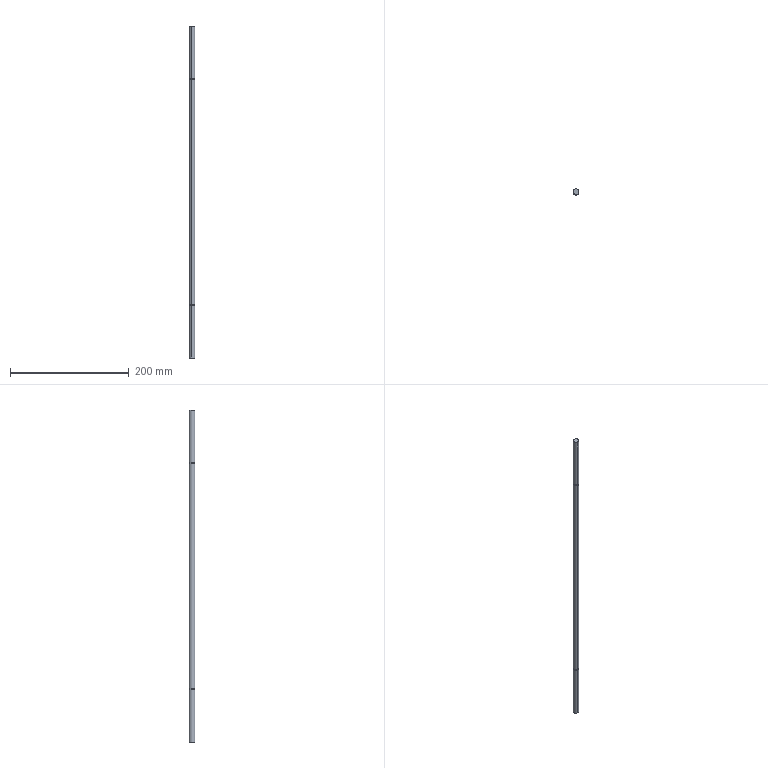Component | SolidWorks | FilmGuideRodAxis-1 | 1 solid | 16 faces | box 10 x 10 x 559 mm | volume 43894 mm3 | cylinder 10 | plane 6 | commonest cylinder face diameters 10 x6 9.7 x4
build123d program:
from build123d import *


with BuildPart() as part:
    # Sketch1 → Revolve1 (revolve)
    with BuildSketch(Plane(origin=(0, 0, 0), x_dir=(-1, 0, 0), z_dir=(0, 0, -1)), mode=Mode.PRIVATE) as revolve1_sk:
        Polygon((-279.5, 5), (-279.5, 0), (279.5, 0), (279.5, 5), (191.1, 5), (191.1, 4.85), (190, 4.85), (190, 5), (-190, 5), (-190, 4.85), (-191.1, 4.85), (-191.1, 5), align=None)
    revolve(revolve1_sk.sketch.rotate(Axis((279.5, 0, 0), (-1, 0, 0)), 270), axis=Axis((279.5, 0, 0), (-1, 0, 0)))


solid = part.part

# Placed as in the assembly
solid = solid.moved(Location((376.258, 489.105, 0), (0, 90, 0)))
STEP:
#1=CARTESIAN_POINT('',(14.853,19.443,7.524));
#2=VERTEX_POINT('',#1);
#3=CARTESIAN_POINT('',(14.773,19.069,7.524));
#4=VERTEX_POINT('',#3);
#5=CARTESIAN_POINT('',(14.813,19.256,7.524));
#6=DIRECTION('',(0.,-0.,-1.));
#7=DIRECTION('',(0.2099,0.9777,0.));
#8=AXIS2_PLACEMENT_3D('',#5,#6,#7);
#9=CIRCLE('',#8,0.1909);
#10=EDGE_CURVE('',#2,#4,#9,.T.);
#11=ORIENTED_EDGE('',*,*,#10,.T.);
#12=CARTESIAN_POINT('',(14.773,19.069,7.48));
#13=VERTEX_POINT('',#12);
#14=CARTESIAN_POINT('',(14.773,19.069,11.004));
#15=DIRECTION('',(0.,-0.,-1.));
#16=VECTOR('',#15,39.37);
#17=LINE('',#14,#16);
#18=EDGE_CURVE('',#4,#13,#17,.T.);
#19=ORIENTED_EDGE('',*,*,#18,.T.);
#20=CARTESIAN_POINT('',(14.853,19.443,7.48));
#21=VERTEX_POINT('',#20);
#22=CARTESIAN_POINT('',(14.813,19.256,7.48));
#23=DIRECTION('',(0.,-0.,-1.));
#24=DIRECTION('',(0.2099,0.9777,0.));
#25=AXIS2_PLACEMENT_3D('',#22,#23,#24);
#26=CIRCLE('',#25,0.1909);
#27=EDGE_CURVE('',#21,#13,#26,.T.);
#28=ORIENTED_EDGE('',*,*,#27,.F.);
#29=CARTESIAN_POINT('',(14.853,19.443,11.004));
#30=DIRECTION('',(0.,-0.,-1.));
#31=VECTOR('',#30,39.37);
#32=LINE('',#29,#31);
#33=EDGE_CURVE('',#2,#21,#32,.T.);
#34=ORIENTED_EDGE('',*,*,#33,.F.);
#35=EDGE_LOOP('',(#11,#19,#28,#34));
#36=FACE_OUTER_BOUND('',#35,.T.);
#37=CARTESIAN_POINT('',(14.813,19.256,11.004));
#38=DIRECTION('',(0.,-0.,-1.));
#39=DIRECTION('',(0.2099,0.9777,0.));
#40=AXIS2_PLACEMENT_3D('',#37,#38,#39);
#41=CYLINDRICAL_SURFACE('',#40,0.1909);
#42=ADVANCED_FACE('',(#36),#41,.T.);
#43=CARTESIAN_POINT('',(14.855,19.449,7.48));
#44=VERTEX_POINT('',#43);
#45=CARTESIAN_POINT('',(14.772,19.064,7.48));
#46=VERTEX_POINT('',#45);
#47=CARTESIAN_POINT('',(14.813,19.256,7.48));
#48=DIRECTION('',(0.,-0.,-1.));
#49=DIRECTION('',(0.2099,0.9777,0.));
#50=AXIS2_PLACEMENT_3D('',#47,#48,#49);
#51=CIRCLE('',#50,0.1969);
#52=EDGE_CURVE('',#44,#46,#51,.T.);
#53=ORIENTED_EDGE('',*,*,#52,.T.);
#54=CARTESIAN_POINT('',(14.772,19.064,-7.48));
#55=VERTEX_POINT('',#54);
#56=CARTESIAN_POINT('',(14.772,19.064,11.004));
#57=DIRECTION('',(0.,-0.,-1.));
#58=VECTOR('',#57,39.37);
#59=LINE('',#56,#58);
#60=EDGE_CURVE('',#46,#55,#59,.T.);
#61=ORIENTED_EDGE('',*,*,#60,.T.);
#62=CARTESIAN_POINT('',(14.855,19.449,-7.48));
#63=VERTEX_POINT('',#62);
#64=CARTESIAN_POINT('',(14.813,19.256,-7.48));
#65=DIRECTION('',(0.,-0.,-1.));
#66=DIRECTION('',(0.2099,0.9777,0.));
#67=AXIS2_PLACEMENT_3D('',#64,#65,#66);
#68=CIRCLE('',#67,0.1969);
#69=EDGE_CURVE('',#63,#55,#68,.T.);
#70=ORIENTED_EDGE('',*,*,#69,.F.);
#71=CARTESIAN_POINT('',(14.855,19.449,11.004));
#72=DIRECTION('',(0.,-0.,-1.));
#73=VECTOR('',#72,39.37);
#74=LINE('',#71,#73);
#75=EDGE_CURVE('',#44,#63,#74,.T.);
#76=ORIENTED_EDGE('',*,*,#75,.F.);
#77=EDGE_LOOP('',(#53,#61,#70,#76));
#78=FACE_OUTER_BOUND('',#77,.T.);
#79=CARTESIAN_POINT('',(14.813,19.256,11.004));
#80=DIRECTION('',(0.,-0.,-1.));
#81=DIRECTION('',(0.2099,0.9777,0.));
#82=AXIS2_PLACEMENT_3D('',#79,#80,#81);
#83=CYLINDRICAL_SURFACE('',#82,0.1969);
#84=ADVANCED_FACE('',(#78),#83,.T.);
#85=CARTESIAN_POINT('',(14.853,19.443,-7.48));
#86=VERTEX_POINT('',#85);
#87=CARTESIAN_POINT('',(14.773,19.069,-7.48));
#88=VERTEX_POINT('',#87);
#89=CARTESIAN_POINT('',(14.813,19.256,-7.48));
#90=DIRECTION('',(0.,-0.,-1.));
#91=DIRECTION('',(0.2099,0.9777,0.));
#92=AXIS2_PLACEMENT_3D('',#89,#90,#91);
#93=CIRCLE('',#92,0.1909);
#94=EDGE_CURVE('',#86,#88,#93,.T.);
#95=ORIENTED_EDGE('',*,*,#94,.T.);
#96=CARTESIAN_POINT('',(14.773,19.069,-7.524));
#97=VERTEX_POINT('',#96);
#98=CARTESIAN_POINT('',(14.773,19.069,11.004));
#99=DIRECTION('',(0.,-0.,-1.));
#100=VECTOR('',#99,39.37);
#101=LINE('',#98,#100);
#102=EDGE_CURVE('',#88,#97,#101,.T.);
#103=ORIENTED_EDGE('',*,*,#102,.T.);
#104=CARTESIAN_POINT('',(14.853,19.443,-7.524));
#105=VERTEX_POINT('',#104);
#106=CARTESIAN_POINT('',(14.813,19.256,-7.524));
#107=DIRECTION('',(0.,-0.,-1.));
#108=DIRECTION('',(0.2099,0.9777,0.));
#109=AXIS2_PLACEMENT_3D('',#106,#107,#108);
#110=CIRCLE('',#109,0.1909);
#111=EDGE_CURVE('',#105,#97,#110,.T.);
#112=ORIENTED_EDGE('',*,*,#111,.F.);
#113=CARTESIAN_POINT('',(14.853,19.443,11.004));
#114=DIRECTION('',(0.,-0.,-1.));
#115=VECTOR('',#114,39.37);
#116=LINE('',#113,#115);
#117=EDGE_CURVE('',#86,#105,#116,.T.);
#118=ORIENTED_EDGE('',*,*,#117,.F.);
#119=EDGE_LOOP('',(#95,#103,#112,#118));
#120=FACE_OUTER_BOUND('',#119,.T.);
#121=CARTESIAN_POINT('',(14.813,19.256,11.004));
#122=DIRECTION('',(0.,-0.,-1.));
#123=DIRECTION('',(0.2099,0.9777,0.));
#124=AXIS2_PLACEMENT_3D('',#121,#122,#123);
#125=CYLINDRICAL_SURFACE('',#124,0.1909);
#126=ADVANCED_FACE('',(#120),#125,.T.);
#127=CARTESIAN_POINT('',(14.855,19.449,-7.524));
#128=VERTEX_POINT('',#127);
#129=CARTESIAN_POINT('',(14.772,19.064,-7.524));
#130=VERTEX_POINT('',#129);
#131=CARTESIAN_POINT('',(14.813,19.256,-7.524));
#132=DIRECTION('',(0.,-0.,-1.));
#133=DIRECTION('',(0.2099,0.9777,0.));
#134=AXIS2_PLACEMENT_3D('',#131,#132,#133);
#135=CIRCLE('',#134,0.1969);
#136=EDGE_CURVE('',#128,#130,#135,.T.);
#137=ORIENTED_EDGE('',*,*,#136,.T.);
#138=CARTESIAN_POINT('',(14.772,19.064,-11.004));
#139=VERTEX_POINT('',#138);
#140=CARTESIAN_POINT('',(14.772,19.064,11.004));
#141=DIRECTION('',(0.,-0.,-1.));
#142=VECTOR('',#141,39.37);
#143=LINE('',#140,#142);
#144=EDGE_CURVE('',#130,#139,#143,.T.);
#145=ORIENTED_EDGE('',*,*,#144,.T.);
#146=CARTESIAN_POINT('',(14.855,19.449,-11.004));
#147=VERTEX_POINT('',#146);
#148=CARTESIAN_POINT('',(14.813,19.256,-11.004));
#149=DIRECTION('',(0.,-0.,-1.));
#150=DIRECTION('',(0.2099,0.9777,0.));
#151=AXIS2_PLACEMENT_3D('',#148,#149,#150);
#152=CIRCLE('',#151,0.1969);
#153=EDGE_CURVE('',#147,#139,#152,.T.);
#154=ORIENTED_EDGE('',*,*,#153,.F.);
#155=CARTESIAN_POINT('',(14.855,19.449,11.004));
#156=DIRECTION('',(0.,-0.,-1.));
#157=VECTOR('',#156,39.37);
#158=LINE('',#155,#157);
#159=EDGE_CURVE('',#128,#147,#158,.T.);
#160=ORIENTED_EDGE('',*,*,#159,.F.);
#161=EDGE_LOOP('',(#137,#145,#154,#160));
#162=FACE_OUTER_BOUND('',#161,.T.);
#163=CARTESIAN_POINT('',(14.813,19.256,11.004));
#164=DIRECTION('',(0.,-0.,-1.));
#165=DIRECTION('',(0.2099,0.9777,0.));
#166=AXIS2_PLACEMENT_3D('',#163,#164,#165);
#167=CYLINDRICAL_SURFACE('',#166,0.1969);
#168=ADVANCED_FACE('',(#162),#167,.T.);
#169=CARTESIAN_POINT('',(14.855,19.449,11.004));
#170=VERTEX_POINT('',#169);
#171=CARTESIAN_POINT('',(14.772,19.064,11.004));
#172=VERTEX_POINT('',#171);
#173=CARTESIAN_POINT('',(14.813,19.256,11.004));
#174=DIRECTION('',(0.,-0.,-1.));
#175=DIRECTION('',(0.2099,0.9777,0.));
#176=AXIS2_PLACEMENT_3D('',#173,#174,#175);
#177=CIRCLE('',#176,0.1969);
#178=EDGE_CURVE('',#170,#172,#177,.T.);
#179=ORIENTED_EDGE('',*,*,#178,.T.);
#180=CARTESIAN_POINT('',(14.772,19.064,7.524));
#181=VERTEX_POINT('',#180);
#182=CARTESIAN_POINT('',(14.772,19.064,11.004));
#183=DIRECTION('',(0.,-0.,-1.));
#184=VECTOR('',#183,39.37);
#185=LINE('',#182,#184);
#186=EDGE_CURVE('',#172,#181,#185,.T.);
#187=ORIENTED_EDGE('',*,*,#186,.T.);
#188=CARTESIAN_POINT('',(14.855,19.449,7.524));
#189=VERTEX_POINT('',#188);
#190=CARTESIAN_POINT('',(14.813,19.256,7.524));
#191=DIRECTION('',(0.,-0.,-1.));
#192=DIRECTION('',(0.2099,0.9777,0.));
#193=AXIS2_PLACEMENT_3D('',#190,#191,#192);
#194=CIRCLE('',#193,0.1969);
#195=EDGE_CURVE('',#189,#181,#194,.T.);
#196=ORIENTED_EDGE('',*,*,#195,.F.);
#197=CARTESIAN_POINT('',(14.855,19.449,11.004));
#198=DIRECTION('',(0.,-0.,-1.));
#199=VECTOR('',#198,39.37);
#200=LINE('',#197,#199);
#201=EDGE_CURVE('',#170,#189,#200,.T.);
#202=ORIENTED_EDGE('',*,*,#201,.F.);
#203=EDGE_LOOP('',(#179,#187,#196,#202));
#204=FACE_OUTER_BOUND('',#203,.T.);
#205=CARTESIAN_POINT('',(14.813,19.256,11.004));
#206=DIRECTION('',(0.,-0.,-1.));
#207=DIRECTION('',(0.2099,0.9777,0.));
#208=AXIS2_PLACEMENT_3D('',#205,#206,#207);
#209=CYLINDRICAL_SURFACE('',#208,0.1969);
#210=ADVANCED_FACE('',(#204),#209,.T.);
#211=ORIENTED_EDGE('',*,*,#186,.F.);
#212=CARTESIAN_POINT('',(14.813,19.256,11.004));
#213=DIRECTION('',(0.,-0.,-1.));
#214=DIRECTION('',(0.2099,0.9777,0.));
#215=AXIS2_PLACEMENT_3D('',#212,#213,#214);
#216=CIRCLE('',#215,0.1969);
#217=EDGE_CURVE('',#172,#170,#216,.T.);
#218=ORIENTED_EDGE('',*,*,#217,.T.);
#219=ORIENTED_EDGE('',*,*,#201,.T.);
#220=CARTESIAN_POINT('',(14.813,19.256,7.524));
#221=DIRECTION('',(0.,-0.,-1.));
#222=DIRECTION('',(0.2099,0.9777,0.));
#223=AXIS2_PLACEMENT_3D('',#220,#221,#222);
#224=CIRCLE('',#223,0.1969);
#225=EDGE_CURVE('',#181,#189,#224,.T.);
#226=ORIENTED_EDGE('',*,*,#225,.F.);
#227=EDGE_LOOP('',(#211,#218,#219,#226));
#228=FACE_OUTER_BOUND('',#227,.T.);
#229=CARTESIAN_POINT('',(14.813,19.256,11.004));
#230=DIRECTION('',(0.,-0.,-1.));
#231=DIRECTION('',(0.2099,0.9777,0.));
#232=AXIS2_PLACEMENT_3D('',#229,#230,#231);
#233=CYLINDRICAL_SURFACE('',#232,0.1969);
#234=ADVANCED_FACE('',(#228),#233,.T.);
#235=ORIENTED_EDGE('',*,*,#178,.F.);
#236=ORIENTED_EDGE('',*,*,#217,.F.);
#237=EDGE_LOOP('',(#235,#236));
#238=FACE_OUTER_BOUND('',#237,.T.);
#239=CARTESIAN_POINT('',(15.006,19.215,11.004));
#240=DIRECTION('',(-0.,0.,1.));
#241=DIRECTION('',(-0.2099,-0.9777,0.));
#242=AXIS2_PLACEMENT_3D('',#239,#240,#241);
#243=PLANE('',#242);
#244=ADVANCED_FACE('',(#238),#243,.T.);
#245=ORIENTED_EDGE('',*,*,#153,.T.);
#246=CARTESIAN_POINT('',(14.813,19.256,-11.004));
#247=DIRECTION('',(0.,-0.,-1.));
#248=DIRECTION('',(0.2099,0.9777,0.));
#249=AXIS2_PLACEMENT_3D('',#246,#247,#248);
#250=CIRCLE('',#249,0.1969);
#251=EDGE_CURVE('',#139,#147,#250,.T.);
#252=ORIENTED_EDGE('',*,*,#251,.T.);
#253=EDGE_LOOP('',(#245,#252));
#254=FACE_OUTER_BOUND('',#253,.T.);
#255=CARTESIAN_POINT('',(14.813,19.256,-11.004));
#256=DIRECTION('',(0.,-0.,-1.));
#257=DIRECTION('',(0.2099,0.9777,0.));
#258=AXIS2_PLACEMENT_3D('',#255,#256,#257);
#259=PLANE('',#258);
#260=ADVANCED_FACE('',(#254),#259,.T.);
#261=ORIENTED_EDGE('',*,*,#144,.F.);
#262=CARTESIAN_POINT('',(14.813,19.256,-7.524));
#263=DIRECTION('',(0.,-0.,-1.));
#264=DIRECTION('',(0.2099,0.9777,0.));
#265=AXIS2_PLACEMENT_3D('',#262,#263,#264);
#266=CIRCLE('',#265,0.1969);
#267=EDGE_CURVE('',#130,#128,#266,.T.);
#268=ORIENTED_EDGE('',*,*,#267,.T.);
#269=ORIENTED_EDGE('',*,*,#159,.T.);
#270=ORIENTED_EDGE('',*,*,#251,.F.);
#271=EDGE_LOOP('',(#261,#268,#269,#270));
#272=FACE_OUTER_BOUND('',#271,.T.);
#273=CARTESIAN_POINT('',(14.813,19.256,11.004));
#274=DIRECTION('',(0.,-0.,-1.));
#275=DIRECTION('',(0.2099,0.9777,0.));
#276=AXIS2_PLACEMENT_3D('',#273,#274,#275);
#277=CYLINDRICAL_SURFACE('',#276,0.1969);
#278=ADVANCED_FACE('',(#272),#277,.T.);
#279=ORIENTED_EDGE('',*,*,#111,.T.);
#280=CARTESIAN_POINT('',(14.813,19.256,-7.524));
#281=DIRECTION('',(0.,-0.,-1.));
#282=DIRECTION('',(0.2099,0.9777,0.));
#283=AXIS2_PLACEMENT_3D('',#280,#281,#282);
#284=CIRCLE('',#283,0.1909);
#285=EDGE_CURVE('',#97,#105,#284,.T.);
#286=ORIENTED_EDGE('',*,*,#285,.T.);
#287=EDGE_LOOP('',(#279,#286));
#288=FACE_BOUND('',#287,.T.);
#289=ORIENTED_EDGE('',*,*,#136,.F.);
#290=ORIENTED_EDGE('',*,*,#267,.F.);
#291=EDGE_LOOP('',(#289,#290));
#292=FACE_OUTER_BOUND('',#291,.T.);
#293=CARTESIAN_POINT('',(15.006,19.215,-7.524));
#294=DIRECTION('',(-0.,0.,1.));
#295=DIRECTION('',(-0.2099,-0.9777,0.));
#296=AXIS2_PLACEMENT_3D('',#293,#294,#295);
#297=PLANE('',#296);
#298=ADVANCED_FACE('',(#288,#292),#297,.T.);
#299=ORIENTED_EDGE('',*,*,#102,.F.);
#300=CARTESIAN_POINT('',(14.813,19.256,-7.48));
#301=DIRECTION('',(0.,-0.,-1.));
#302=DIRECTION('',(0.2099,0.9777,0.));
#303=AXIS2_PLACEMENT_3D('',#300,#301,#302);
#304=CIRCLE('',#303,0.1909);
#305=EDGE_CURVE('',#88,#86,#304,.T.);
#306=ORIENTED_EDGE('',*,*,#305,.T.);
#307=ORIENTED_EDGE('',*,*,#117,.T.);
#308=ORIENTED_EDGE('',*,*,#285,.F.);
#309=EDGE_LOOP('',(#299,#306,#307,#308));
#310=FACE_OUTER_BOUND('',#309,.T.);
#311=CARTESIAN_POINT('',(14.813,19.256,11.004));
#312=DIRECTION('',(0.,-0.,-1.));
#313=DIRECTION('',(0.2099,0.9777,0.));
#314=AXIS2_PLACEMENT_3D('',#311,#312,#313);
#315=CYLINDRICAL_SURFACE('',#314,0.1909);
#316=ADVANCED_FACE('',(#310),#315,.T.);
#317=ORIENTED_EDGE('',*,*,#69,.T.);
#318=CARTESIAN_POINT('',(14.813,19.256,-7.48));
#319=DIRECTION('',(0.,-0.,-1.));
#320=DIRECTION('',(0.2099,0.9777,0.));
#321=AXIS2_PLACEMENT_3D('',#318,#319,#320);
#322=CIRCLE('',#321,0.1969);
#323=EDGE_CURVE('',#55,#63,#322,.T.);
#324=ORIENTED_EDGE('',*,*,#323,.T.);
#325=EDGE_LOOP('',(#317,#324));
#326=FACE_OUTER_BOUND('',#325,.T.);
#327=ORIENTED_EDGE('',*,*,#94,.F.);
#328=ORIENTED_EDGE('',*,*,#305,.F.);
#329=EDGE_LOOP('',(#327,#328));
#330=FACE_BOUND('',#329,.T.);
#331=CARTESIAN_POINT('',(15.,19.216,-7.48));
#332=DIRECTION('',(0.,-0.,-1.));
#333=DIRECTION('',(0.2099,0.9777,0.));
#334=AXIS2_PLACEMENT_3D('',#331,#332,#333);
#335=PLANE('',#334);
#336=ADVANCED_FACE('',(#326,#330),#335,.T.);
#337=ORIENTED_EDGE('',*,*,#60,.F.);
#338=CARTESIAN_POINT('',(14.813,19.256,7.48));
#339=DIRECTION('',(0.,-0.,-1.));
#340=DIRECTION('',(0.2099,0.9777,0.));
#341=AXIS2_PLACEMENT_3D('',#338,#339,#340);
#342=CIRCLE('',#341,0.1969);
#343=EDGE_CURVE('',#46,#44,#342,.T.);
#344=ORIENTED_EDGE('',*,*,#343,.T.);
#345=ORIENTED_EDGE('',*,*,#75,.T.);
#346=ORIENTED_EDGE('',*,*,#323,.F.);
#347=EDGE_LOOP('',(#337,#344,#345,#346));
#348=FACE_OUTER_BOUND('',#347,.T.);
#349=CARTESIAN_POINT('',(14.813,19.256,11.004));
#350=DIRECTION('',(0.,-0.,-1.));
#351=DIRECTION('',(0.2099,0.9777,0.));
#352=AXIS2_PLACEMENT_3D('',#349,#350,#351);
#353=CYLINDRICAL_SURFACE('',#352,0.1969);
#354=ADVANCED_FACE('',(#348),#353,.T.);
#355=ORIENTED_EDGE('',*,*,#27,.T.);
#356=CARTESIAN_POINT('',(14.813,19.256,7.48));
#357=DIRECTION('',(0.,-0.,-1.));
#358=DIRECTION('',(0.2099,0.9777,0.));
#359=AXIS2_PLACEMENT_3D('',#356,#357,#358);
#360=CIRCLE('',#359,0.1909);
#361=EDGE_CURVE('',#13,#21,#360,.T.);
#362=ORIENTED_EDGE('',*,*,#361,.T.);
#363=EDGE_LOOP('',(#355,#362));
#364=FACE_BOUND('',#363,.T.);
#365=ORIENTED_EDGE('',*,*,#52,.F.);
#366=ORIENTED_EDGE('',*,*,#343,.F.);
#367=EDGE_LOOP('',(#365,#366));
#368=FACE_OUTER_BOUND('',#367,.T.);
#369=CARTESIAN_POINT('',(15.006,19.215,7.48));
#370=DIRECTION('',(-0.,0.,1.));
#371=DIRECTION('',(-0.2099,-0.9777,0.));
#372=AXIS2_PLACEMENT_3D('',#369,#370,#371);
#373=PLANE('',#372);
#374=ADVANCED_FACE('',(#364,#368),#373,.T.);
#375=ORIENTED_EDGE('',*,*,#18,.F.);
#376=CARTESIAN_POINT('',(14.813,19.256,7.524));
#377=DIRECTION('',(0.,-0.,-1.));
#378=DIRECTION('',(0.2099,0.9777,0.));
#379=AXIS2_PLACEMENT_3D('',#376,#377,#378);
#380=CIRCLE('',#379,0.1909);
#381=EDGE_CURVE('',#4,#2,#380,.T.);
#382=ORIENTED_EDGE('',*,*,#381,.T.);
#383=ORIENTED_EDGE('',*,*,#33,.T.);
#384=ORIENTED_EDGE('',*,*,#361,.F.);
#385=EDGE_LOOP('',(#375,#382,#383,#384));
#386=FACE_OUTER_BOUND('',#385,.T.);
#387=CARTESIAN_POINT('',(14.813,19.256,11.004));
#388=DIRECTION('',(0.,-0.,-1.));
#389=DIRECTION('',(0.2099,0.9777,0.));
#390=AXIS2_PLACEMENT_3D('',#387,#388,#389);
#391=CYLINDRICAL_SURFACE('',#390,0.1909);
#392=ADVANCED_FACE('',(#386),#391,.T.);
#393=ORIENTED_EDGE('',*,*,#195,.T.);
#394=ORIENTED_EDGE('',*,*,#225,.T.);
#395=EDGE_LOOP('',(#393,#394));
#396=FACE_OUTER_BOUND('',#395,.T.);
#397=ORIENTED_EDGE('',*,*,#10,.F.);
#398=ORIENTED_EDGE('',*,*,#381,.F.);
#399=EDGE_LOOP('',(#397,#398));
#400=FACE_BOUND('',#399,.T.);
#401=CARTESIAN_POINT('',(15.,19.216,7.524));
#402=DIRECTION('',(0.,-0.,-1.));
#403=DIRECTION('',(0.2099,0.9777,0.));
#404=AXIS2_PLACEMENT_3D('',#401,#402,#403);
#405=PLANE('',#404);
#406=ADVANCED_FACE('',(#396,#400),#405,.T.);
#407=CLOSED_SHELL('',(#42,#84,#126,#168,#210,#234,#244,#260,#278,#298,#316,#336,#354,#374,#392,#406));
#408=MANIFOLD_SOLID_BREP('',#407);
#409=CARTESIAN_POINT('',(0.,0.,0.));
#410=DIRECTION('',(0.,0.,1.));
#411=DIRECTION('',(1.,0.,0.));
#412=AXIS2_PLACEMENT_3D('',#409,#410,#411);
#413=(LENGTH_UNIT()NAMED_UNIT(*)SI_UNIT($,.METRE.));
#414=LENGTH_MEASURE_WITH_UNIT(LENGTH_MEASURE(0.0254),#413);
#415=DIMENSIONAL_EXPONENTS(1.,0.,0.,0.,0.,0.,0.);
#416=(CONVERSION_BASED_UNIT('',#414)LENGTH_UNIT()NAMED_UNIT(#415));
#417=UNCERTAINTY_MEASURE_WITH_UNIT(LENGTH_MEASURE(0.00001),#416,'','');
#418=(NAMED_UNIT(*)PLANE_ANGLE_UNIT()SI_UNIT($,.RADIAN.));
#419=(NAMED_UNIT(*)SI_UNIT($,.STERADIAN.)SOLID_ANGLE_UNIT());
#420=(GEOMETRIC_REPRESENTATION_CONTEXT(3)GLOBAL_UNCERTAINTY_ASSIGNED_CONTEXT((#417))GLOBAL_UNIT_ASSIGNED_CONTEXT((#416,#418,#419))REPRESENTATION_CONTEXT('',''));
#421=ADVANCED_BREP_SHAPE_REPRESENTATION('',(#408,#412),#420);
#422=COLOUR_RGB('',0.7922,0.8196,0.9333);
#423=FILL_AREA_STYLE_COLOUR('',#422);
#424=FILL_AREA_STYLE('',(#423));
#425=SURFACE_STYLE_FILL_AREA(#424);
#426=SURFACE_SIDE_STYLE('',(#425));
#427=SURFACE_STYLE_USAGE(.BOTH.,#426);
#428=PRESENTATION_STYLE_ASSIGNMENT((#427));
#429=STYLED_ITEM('',(#428),#408);
#430=(LENGTH_UNIT()NAMED_UNIT(*)SI_UNIT($,.METRE.));
#431=LENGTH_MEASURE_WITH_UNIT(LENGTH_MEASURE(0.0254),#430);
#432=DIMENSIONAL_EXPONENTS(1.,0.,0.,0.,0.,0.,0.);
#433=(CONVERSION_BASED_UNIT('',#431)LENGTH_UNIT()NAMED_UNIT(#432));
#434=UNCERTAINTY_MEASURE_WITH_UNIT(LENGTH_MEASURE(0.00001),#433,'','');
#435=(NAMED_UNIT(*)PLANE_ANGLE_UNIT()SI_UNIT($,.RADIAN.));
#436=(NAMED_UNIT(*)SI_UNIT($,.STERADIAN.)SOLID_ANGLE_UNIT());
#437=(GEOMETRIC_REPRESENTATION_CONTEXT(3)GLOBAL_UNCERTAINTY_ASSIGNED_CONTEXT((#434))GLOBAL_UNIT_ASSIGNED_CONTEXT((#433,#435,#436))REPRESENTATION_CONTEXT('',''));
#438=MECHANICAL_DESIGN_GEOMETRIC_PRESENTATION_REPRESENTATION('',(#429),#437);
#439=PRESENTATION_LAYER_ASSIGNMENT('','',(#429));